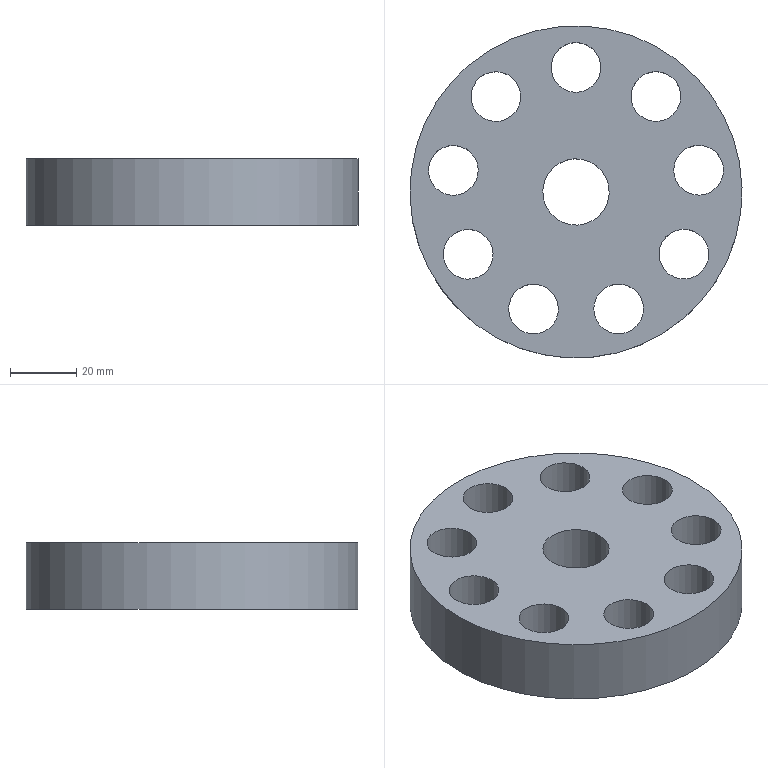Component | NX | CARK1 | 1 solid | 13 faces | box 100 x 100 x 20 mm | volume 118988 mm3 | cylinder 11 | plane 2 | commonest cylinder face diameters 15 x9 20 x1 100 x1
STEP:
#1=CARTESIAN_POINT('',(0.,0.,0.));
#2=DIRECTION('',(0.,0.,1.));
#3=DIRECTION('',(1.,0.,0.));
#4=AXIS2_PLACEMENT_3D('',#1,#2,#3);
#5=CARTESIAN_POINT('',(-1129.876,961.837,201.928));
#6=VERTEX_POINT('',#5);
#7=CARTESIAN_POINT('',(-1123.378,958.091,201.928));
#8=DIRECTION('',(0.,0.,-1.));
#9=DIRECTION('',(-0.8663,0.4995,0.));
#10=AXIS2_PLACEMENT_3D('',#7,#8,#9);
#11=CIRCLE('',#10,7.5);
#12=CARTESIAN_POINT('',(-1123.378,958.091,201.928));
#13=DIRECTION('',(0.,0.,1.));
#14=DIRECTION('',(-0.1743,0.9847,0.));
#15=AXIS2_PLACEMENT_3D('',#12,#13,#14);
#16=CYLINDRICAL_SURFACE('',#15,7.5);
#17=CARTESIAN_POINT('',(7.156,0.));
#18=DIRECTION('',(-1.,0.));
#19=VECTOR('',#18,1.);
#20=LINE('',#17,#19);
#21=(GEOMETRIC_REPRESENTATION_CONTEXT(2)PARAMETRIC_REPRESENTATION_CONTEXT()REPRESENTATION_CONTEXT('',''));
#22=DEFINITIONAL_REPRESENTATION('',(#20),#21);
#23=PCURVE('',#16,#22);
#24=CARTESIAN_POINT('',(-1174.333,980.065,201.928));
#25=DIRECTION('',(0.,0.,-1.));
#26=DIRECTION('',(0.1743,-0.9847,0.));
#27=AXIS2_PLACEMENT_3D('',#24,#25,#26);
#28=PLANE('',#27);
#29=CARTESIAN_POINT('',(30.517,-46.346));
#30=DIRECTION('',(-0.6428,0.766));
#31=AXIS2_PLACEMENT_2D('',#29,#30);
#32=CIRCLE('',#31,7.5);
#33=(GEOMETRIC_REPRESENTATION_CONTEXT(2)PARAMETRIC_REPRESENTATION_CONTEXT()REPRESENTATION_CONTEXT('',''));
#34=DEFINITIONAL_REPRESENTATION('',(#32),#33);
#35=PCURVE('',#28,#34);
#36=SURFACE_CURVE('',#11,(#23,#35),.PCURVE_S1.);
#37=EDGE_CURVE('',#6,#6,#36,.T.);
#38=ORIENTED_EDGE('',*,*,#37,.F.);
#39=CARTESIAN_POINT('',(-1129.876,961.837,221.928));
#40=VERTEX_POINT('',#39);
#41=CARTESIAN_POINT('',(-1129.876,961.837,201.928));
#42=CARTESIAN_POINT('',(-1129.876,961.837,221.928));
#43=B_SPLINE_CURVE_WITH_KNOTS('',1,(#41,#42),.UNSPECIFIED.,.F.,.F.,(2,2),(0.,20.),.PIECEWISE_BEZIER_KNOTS.);
#44=CARTESIAN_POINT('',(7.156,0.));
#45=DIRECTION('',(0.,1.));
#46=VECTOR('',#45,1.);
#47=LINE('',#44,#46);
#48=(GEOMETRIC_REPRESENTATION_CONTEXT(2)PARAMETRIC_REPRESENTATION_CONTEXT()REPRESENTATION_CONTEXT('',''));
#49=DEFINITIONAL_REPRESENTATION('',(#47),#48);
#50=PCURVE('',#16,#49);
#51=CARTESIAN_POINT('',(0.8727,0.));
#52=DIRECTION('',(0.,1.));
#53=VECTOR('',#52,1.);
#54=LINE('',#51,#53);
#55=(GEOMETRIC_REPRESENTATION_CONTEXT(2)PARAMETRIC_REPRESENTATION_CONTEXT()REPRESENTATION_CONTEXT('',''));
#56=DEFINITIONAL_REPRESENTATION('',(#54),#55);
#57=PCURVE('',#16,#56);
#58=SEAM_CURVE('',#43,(#50,#57),.PCURVE_S1.);
#59=EDGE_CURVE('',#6,#40,#58,.T.);
#60=ORIENTED_EDGE('',*,*,#59,.T.);
#61=CARTESIAN_POINT('',(-1123.378,958.091,221.928));
#62=DIRECTION('',(0.,0.,-1.));
#63=DIRECTION('',(-0.8663,0.4995,0.));
#64=AXIS2_PLACEMENT_3D('',#61,#62,#63);
#65=CIRCLE('',#64,7.5);
#66=CARTESIAN_POINT('',(7.156,20.));
#67=DIRECTION('',(-1.,0.));
#68=VECTOR('',#67,1.);
#69=LINE('',#66,#68);
#70=(GEOMETRIC_REPRESENTATION_CONTEXT(2)PARAMETRIC_REPRESENTATION_CONTEXT()REPRESENTATION_CONTEXT('',''));
#71=DEFINITIONAL_REPRESENTATION('',(#69),#70);
#72=PCURVE('',#16,#71);
#73=CARTESIAN_POINT('',(-1174.333,980.065,221.928));
#74=DIRECTION('',(0.,0.,-1.));
#75=DIRECTION('',(0.1743,-0.9847,0.));
#76=AXIS2_PLACEMENT_3D('',#73,#74,#75);
#77=PLANE('',#76);
#78=CARTESIAN_POINT('',(30.517,-46.346));
#79=DIRECTION('',(-0.6428,0.766));
#80=AXIS2_PLACEMENT_2D('',#78,#79);
#81=CIRCLE('',#80,7.5);
#82=(GEOMETRIC_REPRESENTATION_CONTEXT(2)PARAMETRIC_REPRESENTATION_CONTEXT()REPRESENTATION_CONTEXT('',''));
#83=DEFINITIONAL_REPRESENTATION('',(#81),#82);
#84=PCURVE('',#77,#83);
#85=SURFACE_CURVE('',#65,(#72,#84),.PCURVE_S1.);
#86=EDGE_CURVE('',#40,#40,#85,.T.);
#87=ORIENTED_EDGE('',*,*,#86,.T.);
#88=ORIENTED_EDGE('',*,*,#59,.F.);
#89=EDGE_LOOP('',(#38,#60,#87,#88));
#90=FACE_BOUND('',#89,.F.);
#91=ADVANCED_FACE('',(#90),#16,.F.);
#92=CARTESIAN_POINT('',(-1136.597,999.814,201.928));
#93=VERTEX_POINT('',#92);
#94=CARTESIAN_POINT('',(-1131.78,1005.562,201.928));
#95=DIRECTION('',(0.,0.,-1.));
#96=DIRECTION('',(-0.6423,-0.7665,0.));
#97=AXIS2_PLACEMENT_3D('',#94,#95,#96);
#98=CIRCLE('',#97,7.5);
#99=CARTESIAN_POINT('',(-1131.78,1005.562,201.928));
#100=DIRECTION('',(0.,0.,1.));
#101=DIRECTION('',(-0.1743,0.9847,0.));
#102=AXIS2_PLACEMENT_3D('',#99,#100,#101);
#103=CYLINDRICAL_SURFACE('',#102,7.5);
#104=CARTESIAN_POINT('',(8.552,0.));
#105=DIRECTION('',(-1.,0.));
#106=VECTOR('',#105,1.);
#107=LINE('',#104,#106);
#108=(GEOMETRIC_REPRESENTATION_CONTEXT(2)PARAMETRIC_REPRESENTATION_CONTEXT()REPRESENTATION_CONTEXT('',''));
#109=DEFINITIONAL_REPRESENTATION('',(#107),#108);
#110=PCURVE('',#103,#109);
#111=CARTESIAN_POINT('',(-17.692,-46.346));
#112=DIRECTION('',(0.6428,0.766));
#113=AXIS2_PLACEMENT_2D('',#111,#112);
#114=CIRCLE('',#113,7.5);
#115=(GEOMETRIC_REPRESENTATION_CONTEXT(2)PARAMETRIC_REPRESENTATION_CONTEXT()REPRESENTATION_CONTEXT('',''));
#116=DEFINITIONAL_REPRESENTATION('',(#114),#115);
#117=PCURVE('',#28,#116);
#118=SURFACE_CURVE('',#98,(#110,#117),.PCURVE_S1.);
#119=EDGE_CURVE('',#93,#93,#118,.T.);
#120=ORIENTED_EDGE('',*,*,#119,.F.);
#121=CARTESIAN_POINT('',(-1136.597,999.814,221.928));
#122=VERTEX_POINT('',#121);
#123=CARTESIAN_POINT('',(-1136.597,999.814,201.928));
#124=CARTESIAN_POINT('',(-1136.597,999.814,221.928));
#125=B_SPLINE_CURVE_WITH_KNOTS('',1,(#123,#124),.UNSPECIFIED.,.F.,.F.,(2,2),(0.,20.),.PIECEWISE_BEZIER_KNOTS.);
#126=CARTESIAN_POINT('',(8.552,0.));
#127=DIRECTION('',(0.,1.));
#128=VECTOR('',#127,1.);
#129=LINE('',#126,#128);
#130=(GEOMETRIC_REPRESENTATION_CONTEXT(2)PARAMETRIC_REPRESENTATION_CONTEXT()REPRESENTATION_CONTEXT('',''));
#131=DEFINITIONAL_REPRESENTATION('',(#129),#130);
#132=PCURVE('',#103,#131);
#133=CARTESIAN_POINT('',(2.269,0.));
#134=DIRECTION('',(0.,1.));
#135=VECTOR('',#134,1.);
#136=LINE('',#133,#135);
#137=(GEOMETRIC_REPRESENTATION_CONTEXT(2)PARAMETRIC_REPRESENTATION_CONTEXT()REPRESENTATION_CONTEXT('',''));
#138=DEFINITIONAL_REPRESENTATION('',(#136),#137);
#139=PCURVE('',#103,#138);
#140=SEAM_CURVE('',#125,(#132,#139),.PCURVE_S1.);
#141=EDGE_CURVE('',#93,#122,#140,.T.);
#142=ORIENTED_EDGE('',*,*,#141,.T.);
#143=CARTESIAN_POINT('',(-1131.78,1005.562,221.928));
#144=DIRECTION('',(0.,0.,-1.));
#145=DIRECTION('',(-0.6423,-0.7665,0.));
#146=AXIS2_PLACEMENT_3D('',#143,#144,#145);
#147=CIRCLE('',#146,7.5);
#148=CARTESIAN_POINT('',(8.552,20.));
#149=DIRECTION('',(-1.,0.));
#150=VECTOR('',#149,1.);
#151=LINE('',#148,#150);
#152=(GEOMETRIC_REPRESENTATION_CONTEXT(2)PARAMETRIC_REPRESENTATION_CONTEXT()REPRESENTATION_CONTEXT('',''));
#153=DEFINITIONAL_REPRESENTATION('',(#151),#152);
#154=PCURVE('',#103,#153);
#155=CARTESIAN_POINT('',(-17.692,-46.346));
#156=DIRECTION('',(0.6428,0.766));
#157=AXIS2_PLACEMENT_2D('',#155,#156);
#158=CIRCLE('',#157,7.5);
#159=(GEOMETRIC_REPRESENTATION_CONTEXT(2)PARAMETRIC_REPRESENTATION_CONTEXT()REPRESENTATION_CONTEXT('',''));
#160=DEFINITIONAL_REPRESENTATION('',(#158),#159);
#161=PCURVE('',#77,#160);
#162=SURFACE_CURVE('',#147,(#154,#161),.PCURVE_S1.);
#163=EDGE_CURVE('',#122,#122,#162,.T.);
#164=ORIENTED_EDGE('',*,*,#163,.T.);
#165=ORIENTED_EDGE('',*,*,#141,.F.);
#166=EDGE_LOOP('',(#120,#142,#164,#165));
#167=FACE_BOUND('',#166,.F.);
#168=ADVANCED_FACE('',(#167),#103,.F.);
#169=CARTESIAN_POINT('',(-1145.588,948.636,201.928));
#170=VERTEX_POINT('',#169);
#171=CARTESIAN_POINT('',(-1143.018,941.59,201.928));
#172=DIRECTION('',(0.,0.,-1.));
#173=DIRECTION('',(-0.3426,0.9395,0.));
#174=AXIS2_PLACEMENT_3D('',#171,#172,#173);
#175=CIRCLE('',#174,7.5);
#176=CARTESIAN_POINT('',(-1143.018,941.59,201.928));
#177=DIRECTION('',(0.,0.,1.));
#178=DIRECTION('',(-0.1743,0.9847,0.));
#179=AXIS2_PLACEMENT_3D('',#176,#177,#178);
#180=CYLINDRICAL_SURFACE('',#179,7.5);
#181=CARTESIAN_POINT('',(6.458,0.));
#182=DIRECTION('',(-1.,0.));
#183=VECTOR('',#182,1.);
#184=LINE('',#181,#183);
#185=(GEOMETRIC_REPRESENTATION_CONTEXT(2)PARAMETRIC_REPRESENTATION_CONTEXT()REPRESENTATION_CONTEXT('',''));
#186=DEFINITIONAL_REPRESENTATION('',(#184),#185);
#187=PCURVE('',#180,#186);
#188=CARTESIAN_POINT('',(43.343,-24.131));
#189=DIRECTION('',(-0.9848,0.1736));
#190=AXIS2_PLACEMENT_2D('',#188,#189);
#191=CIRCLE('',#190,7.5);
#192=(GEOMETRIC_REPRESENTATION_CONTEXT(2)PARAMETRIC_REPRESENTATION_CONTEXT()REPRESENTATION_CONTEXT('',''));
#193=DEFINITIONAL_REPRESENTATION('',(#191),#192);
#194=PCURVE('',#28,#193);
#195=SURFACE_CURVE('',#175,(#187,#194),.PCURVE_S1.);
#196=EDGE_CURVE('',#170,#170,#195,.T.);
#197=ORIENTED_EDGE('',*,*,#196,.F.);
#198=CARTESIAN_POINT('',(-1145.588,948.636,221.928));
#199=VERTEX_POINT('',#198);
#200=CARTESIAN_POINT('',(-1145.588,948.636,201.928));
#201=CARTESIAN_POINT('',(-1145.588,948.636,221.928));
#202=B_SPLINE_CURVE_WITH_KNOTS('',1,(#200,#201),.UNSPECIFIED.,.F.,.F.,(2,2),(0.,20.),.PIECEWISE_BEZIER_KNOTS.);
#203=CARTESIAN_POINT('',(6.458,0.));
#204=DIRECTION('',(0.,1.));
#205=VECTOR('',#204,1.);
#206=LINE('',#203,#205);
#207=(GEOMETRIC_REPRESENTATION_CONTEXT(2)PARAMETRIC_REPRESENTATION_CONTEXT()REPRESENTATION_CONTEXT('',''));
#208=DEFINITIONAL_REPRESENTATION('',(#206),#207);
#209=PCURVE('',#180,#208);
#210=CARTESIAN_POINT('',(0.1745,0.));
#211=DIRECTION('',(0.,1.));
#212=VECTOR('',#211,1.);
#213=LINE('',#210,#212);
#214=(GEOMETRIC_REPRESENTATION_CONTEXT(2)PARAMETRIC_REPRESENTATION_CONTEXT()REPRESENTATION_CONTEXT('',''));
#215=DEFINITIONAL_REPRESENTATION('',(#213),#214);
#216=PCURVE('',#180,#215);
#217=SEAM_CURVE('',#202,(#209,#216),.PCURVE_S1.);
#218=EDGE_CURVE('',#170,#199,#217,.T.);
#219=ORIENTED_EDGE('',*,*,#218,.T.);
#220=CARTESIAN_POINT('',(-1143.018,941.59,221.928));
#221=DIRECTION('',(0.,0.,-1.));
#222=DIRECTION('',(-0.3426,0.9395,0.));
#223=AXIS2_PLACEMENT_3D('',#220,#221,#222);
#224=CIRCLE('',#223,7.5);
#225=CARTESIAN_POINT('',(6.458,20.));
#226=DIRECTION('',(-1.,0.));
#227=VECTOR('',#226,1.);
#228=LINE('',#225,#227);
#229=(GEOMETRIC_REPRESENTATION_CONTEXT(2)PARAMETRIC_REPRESENTATION_CONTEXT()REPRESENTATION_CONTEXT('',''));
#230=DEFINITIONAL_REPRESENTATION('',(#228),#229);
#231=PCURVE('',#180,#230);
#232=CARTESIAN_POINT('',(43.343,-24.131));
#233=DIRECTION('',(-0.9848,0.1736));
#234=AXIS2_PLACEMENT_2D('',#232,#233);
#235=CIRCLE('',#234,7.5);
#236=(GEOMETRIC_REPRESENTATION_CONTEXT(2)PARAMETRIC_REPRESENTATION_CONTEXT()REPRESENTATION_CONTEXT('',''));
#237=DEFINITIONAL_REPRESENTATION('',(#235),#236);
#238=PCURVE('',#77,#237);
#239=SURFACE_CURVE('',#224,(#231,#238),.PCURVE_S1.);
#240=EDGE_CURVE('',#199,#199,#239,.T.);
#241=ORIENTED_EDGE('',*,*,#240,.T.);
#242=ORIENTED_EDGE('',*,*,#218,.F.);
#243=EDGE_LOOP('',(#197,#219,#241,#242));
#244=FACE_BOUND('',#243,.F.);
#245=ADVANCED_FACE('',(#244),#180,.F.);
#246=CARTESIAN_POINT('',(-1155.885,1006.821,201.928));
#247=VERTEX_POINT('',#246);
#248=CARTESIAN_POINT('',(-1155.89,1014.321,201.928));
#249=DIRECTION('',(0.,0.,-1.));
#250=DIRECTION('',(0.0006313,-1.,0.));
#251=AXIS2_PLACEMENT_3D('',#248,#249,#250);
#252=CIRCLE('',#251,7.5);
#253=CARTESIAN_POINT('',(-1155.89,1014.321,201.928));
#254=DIRECTION('',(0.,0.,1.));
#255=DIRECTION('',(-0.1743,0.9847,0.));
#256=AXIS2_PLACEMENT_3D('',#253,#254,#255);
#257=CYLINDRICAL_SURFACE('',#256,7.5);
#258=CARTESIAN_POINT('',(9.25,0.));
#259=DIRECTION('',(-1.,0.));
#260=VECTOR('',#259,1.);
#261=LINE('',#258,#260);
#262=(GEOMETRIC_REPRESENTATION_CONTEXT(2)PARAMETRIC_REPRESENTATION_CONTEXT()REPRESENTATION_CONTEXT('',''));
#263=DEFINITIONAL_REPRESENTATION('',(#261),#262);
#264=PCURVE('',#257,#263);
#265=CARTESIAN_POINT('',(-30.517,-24.131));
#266=DIRECTION('',(0.9848,0.1736));
#267=AXIS2_PLACEMENT_2D('',#265,#266);
#268=CIRCLE('',#267,7.5);
#269=(GEOMETRIC_REPRESENTATION_CONTEXT(2)PARAMETRIC_REPRESENTATION_CONTEXT()REPRESENTATION_CONTEXT('',''));
#270=DEFINITIONAL_REPRESENTATION('',(#268),#269);
#271=PCURVE('',#28,#270);
#272=SURFACE_CURVE('',#252,(#264,#271),.PCURVE_S1.);
#273=EDGE_CURVE('',#247,#247,#272,.T.);
#274=ORIENTED_EDGE('',*,*,#273,.F.);
#275=CARTESIAN_POINT('',(-1155.885,1006.821,221.928));
#276=VERTEX_POINT('',#275);
#277=CARTESIAN_POINT('',(-1155.885,1006.821,201.928));
#278=CARTESIAN_POINT('',(-1155.885,1006.821,221.928));
#279=B_SPLINE_CURVE_WITH_KNOTS('',1,(#277,#278),.UNSPECIFIED.,.F.,.F.,(2,2),(0.,20.),.PIECEWISE_BEZIER_KNOTS.);
#280=CARTESIAN_POINT('',(9.25,0.));
#281=DIRECTION('',(0.,1.));
#282=VECTOR('',#281,1.);
#283=LINE('',#280,#282);
#284=(GEOMETRIC_REPRESENTATION_CONTEXT(2)PARAMETRIC_REPRESENTATION_CONTEXT()REPRESENTATION_CONTEXT('',''));
#285=DEFINITIONAL_REPRESENTATION('',(#283),#284);
#286=PCURVE('',#257,#285);
#287=CARTESIAN_POINT('',(2.967,0.));
#288=DIRECTION('',(0.,1.));
#289=VECTOR('',#288,1.);
#290=LINE('',#287,#289);
#291=(GEOMETRIC_REPRESENTATION_CONTEXT(2)PARAMETRIC_REPRESENTATION_CONTEXT()REPRESENTATION_CONTEXT('',''));
#292=DEFINITIONAL_REPRESENTATION('',(#290),#291);
#293=PCURVE('',#257,#292);
#294=SEAM_CURVE('',#279,(#286,#293),.PCURVE_S1.);
#295=EDGE_CURVE('',#247,#276,#294,.T.);
#296=ORIENTED_EDGE('',*,*,#295,.T.);
#297=CARTESIAN_POINT('',(-1155.89,1014.321,221.928));
#298=DIRECTION('',(0.,0.,-1.));
#299=DIRECTION('',(0.0006313,-1.,0.));
#300=AXIS2_PLACEMENT_3D('',#297,#298,#299);
#301=CIRCLE('',#300,7.5);
#302=CARTESIAN_POINT('',(9.25,20.));
#303=DIRECTION('',(-1.,0.));
#304=VECTOR('',#303,1.);
#305=LINE('',#302,#304);
#306=(GEOMETRIC_REPRESENTATION_CONTEXT(2)PARAMETRIC_REPRESENTATION_CONTEXT()REPRESENTATION_CONTEXT('',''));
#307=DEFINITIONAL_REPRESENTATION('',(#305),#306);
#308=PCURVE('',#257,#307);
#309=CARTESIAN_POINT('',(-30.517,-24.131));
#310=DIRECTION('',(0.9848,0.1736));
#311=AXIS2_PLACEMENT_2D('',#309,#310);
#312=CIRCLE('',#311,7.5);
#313=(GEOMETRIC_REPRESENTATION_CONTEXT(2)PARAMETRIC_REPRESENTATION_CONTEXT()REPRESENTATION_CONTEXT('',''));
#314=DEFINITIONAL_REPRESENTATION('',(#312),#313);
#315=PCURVE('',#77,#314);
#316=SURFACE_CURVE('',#301,(#308,#315),.PCURVE_S1.);
#317=EDGE_CURVE('',#276,#276,#316,.T.);
#318=ORIENTED_EDGE('',*,*,#317,.T.);
#319=ORIENTED_EDGE('',*,*,#295,.F.);
#320=EDGE_LOOP('',(#274,#296,#318,#319));
#321=FACE_BOUND('',#320,.F.);
#322=ADVANCED_FACE('',(#321),#257,.F.);
#323=CARTESIAN_POINT('',(-1165.713,975.078,201.928));
#324=VERTEX_POINT('',#323);
#325=CARTESIAN_POINT('',(-1155.866,976.821,201.928));
#326=DIRECTION('',(0.,0.,-1.));
#327=DIRECTION('',(-0.9847,-0.1743,0.));
#328=AXIS2_PLACEMENT_3D('',#325,#326,#327);
#329=CIRCLE('',#328,10.);
#330=CARTESIAN_POINT('',(-1155.866,976.821,201.928));
#331=DIRECTION('',(0.,0.,1.));
#332=DIRECTION('',(-0.1743,0.9847,0.));
#333=AXIS2_PLACEMENT_3D('',#330,#331,#332);
#334=CYLINDRICAL_SURFACE('',#333,10.);
#335=CARTESIAN_POINT('',(7.854,0.));
#336=DIRECTION('',(-1.,0.));
#337=VECTOR('',#336,1.);
#338=LINE('',#335,#337);
#339=(GEOMETRIC_REPRESENTATION_CONTEXT(2)PARAMETRIC_REPRESENTATION_CONTEXT()REPRESENTATION_CONTEXT('',''));
#340=DEFINITIONAL_REPRESENTATION('',(#338),#339);
#341=PCURVE('',#334,#340);
#342=CARTESIAN_POINT('',(6.413,-17.619));
#343=DIRECTION('',(0.,1.));
#344=AXIS2_PLACEMENT_2D('',#342,#343);
#345=CIRCLE('',#344,10.);
#346=(GEOMETRIC_REPRESENTATION_CONTEXT(2)PARAMETRIC_REPRESENTATION_CONTEXT()REPRESENTATION_CONTEXT('',''));
#347=DEFINITIONAL_REPRESENTATION('',(#345),#346);
#348=PCURVE('',#28,#347);
#349=SURFACE_CURVE('',#329,(#341,#348),.PCURVE_S1.);
#350=EDGE_CURVE('',#324,#324,#349,.T.);
#351=ORIENTED_EDGE('',*,*,#350,.F.);
#352=CARTESIAN_POINT('',(-1165.713,975.078,221.928));
#353=VERTEX_POINT('',#352);
#354=CARTESIAN_POINT('',(-1165.713,975.078,201.928));
#355=CARTESIAN_POINT('',(-1165.713,975.078,221.928));
#356=B_SPLINE_CURVE_WITH_KNOTS('',1,(#354,#355),.UNSPECIFIED.,.F.,.F.,(2,2),(0.,20.),.PIECEWISE_BEZIER_KNOTS.);
#357=CARTESIAN_POINT('',(7.854,0.));
#358=DIRECTION('',(0.,1.));
#359=VECTOR('',#358,1.);
#360=LINE('',#357,#359);
#361=(GEOMETRIC_REPRESENTATION_CONTEXT(2)PARAMETRIC_REPRESENTATION_CONTEXT()REPRESENTATION_CONTEXT('',''));
#362=DEFINITIONAL_REPRESENTATION('',(#360),#361);
#363=PCURVE('',#334,#362);
#364=CARTESIAN_POINT('',(1.571,0.));
#365=DIRECTION('',(0.,1.));
#366=VECTOR('',#365,1.);
#367=LINE('',#364,#366);
#368=(GEOMETRIC_REPRESENTATION_CONTEXT(2)PARAMETRIC_REPRESENTATION_CONTEXT()REPRESENTATION_CONTEXT('',''));
#369=DEFINITIONAL_REPRESENTATION('',(#367),#368);
#370=PCURVE('',#334,#369);
#371=SEAM_CURVE('',#356,(#363,#370),.PCURVE_S1.);
#372=EDGE_CURVE('',#324,#353,#371,.T.);
#373=ORIENTED_EDGE('',*,*,#372,.T.);
#374=CARTESIAN_POINT('',(-1155.866,976.821,221.928));
#375=DIRECTION('',(0.,0.,-1.));
#376=DIRECTION('',(-0.9847,-0.1743,0.));
#377=AXIS2_PLACEMENT_3D('',#374,#375,#376);
#378=CIRCLE('',#377,10.);
#379=CARTESIAN_POINT('',(7.854,20.));
#380=DIRECTION('',(-1.,0.));
#381=VECTOR('',#380,1.);
#382=LINE('',#379,#381);
#383=(GEOMETRIC_REPRESENTATION_CONTEXT(2)PARAMETRIC_REPRESENTATION_CONTEXT()REPRESENTATION_CONTEXT('',''));
#384=DEFINITIONAL_REPRESENTATION('',(#382),#383);
#385=PCURVE('',#334,#384);
#386=CARTESIAN_POINT('',(6.413,-17.619));
#387=DIRECTION('',(0.,1.));
#388=AXIS2_PLACEMENT_2D('',#386,#387);
#389=CIRCLE('',#388,10.);
#390=(GEOMETRIC_REPRESENTATION_CONTEXT(2)PARAMETRIC_REPRESENTATION_CONTEXT()REPRESENTATION_CONTEXT('',''));
#391=DEFINITIONAL_REPRESENTATION('',(#389),#390);
#392=PCURVE('',#77,#391);
#393=SURFACE_CURVE('',#378,(#385,#392),.PCURVE_S1.);
#394=EDGE_CURVE('',#353,#353,#393,.T.);
#395=ORIENTED_EDGE('',*,*,#394,.T.);
#396=ORIENTED_EDGE('',*,*,#372,.F.);
#397=EDGE_LOOP('',(#351,#373,#395,#396));
#398=FACE_BOUND('',#397,.F.);
#399=ADVANCED_FACE('',(#398),#334,.F.);
#400=CARTESIAN_POINT('',(-1166.109,948.623,201.928));
#401=VERTEX_POINT('',#400);
#402=CARTESIAN_POINT('',(-1168.67,941.574,201.928));
#403=DIRECTION('',(0.,0.,-1.));
#404=DIRECTION('',(0.3414,0.9399,0.));
#405=AXIS2_PLACEMENT_3D('',#402,#403,#404);
#406=CIRCLE('',#405,7.5);
#407=CARTESIAN_POINT('',(-1168.67,941.574,201.928));
#408=DIRECTION('',(0.,0.,1.));
#409=DIRECTION('',(-0.1743,0.9847,0.));
#410=AXIS2_PLACEMENT_3D('',#407,#408,#409);
#411=CYLINDRICAL_SURFACE('',#410,7.5);
#412=CARTESIAN_POINT('',(12.043,0.));
#413=DIRECTION('',(-1.,0.));
#414=VECTOR('',#413,1.);
#415=LINE('',#412,#414);
#416=(GEOMETRIC_REPRESENTATION_CONTEXT(2)PARAMETRIC_REPRESENTATION_CONTEXT()REPRESENTATION_CONTEXT('',''));
#417=DEFINITIONAL_REPRESENTATION('',(#415),#416);
#418=PCURVE('',#411,#417);
#419=CARTESIAN_POINT('',(38.889,1.131));
#420=DIRECTION('',(-0.866,-0.5));
#421=AXIS2_PLACEMENT_2D('',#419,#420);
#422=CIRCLE('',#421,7.5);
#423=(GEOMETRIC_REPRESENTATION_CONTEXT(2)PARAMETRIC_REPRESENTATION_CONTEXT()REPRESENTATION_CONTEXT('',''));
#424=DEFINITIONAL_REPRESENTATION('',(#422),#423);
#425=PCURVE('',#28,#424);
#426=SURFACE_CURVE('',#406,(#418,#425),.PCURVE_S1.);
#427=EDGE_CURVE('',#401,#401,#426,.T.);
#428=ORIENTED_EDGE('',*,*,#427,.F.);
#429=CARTESIAN_POINT('',(-1166.109,948.623,221.928));
#430=VERTEX_POINT('',#429);
#431=CARTESIAN_POINT('',(-1166.109,948.623,201.928));
#432=CARTESIAN_POINT('',(-1166.109,948.623,221.928));
#433=B_SPLINE_CURVE_WITH_KNOTS('',1,(#431,#432),.UNSPECIFIED.,.F.,.F.,(2,2),(0.,20.),.PIECEWISE_BEZIER_KNOTS.);
#434=CARTESIAN_POINT('',(12.043,0.));
#435=DIRECTION('',(0.,1.));
#436=VECTOR('',#435,1.);
#437=LINE('',#434,#436);
#438=(GEOMETRIC_REPRESENTATION_CONTEXT(2)PARAMETRIC_REPRESENTATION_CONTEXT()REPRESENTATION_CONTEXT('',''));
#439=DEFINITIONAL_REPRESENTATION('',(#437),#438);
#440=PCURVE('',#411,#439);
#441=CARTESIAN_POINT('',(5.76,0.));
#442=DIRECTION('',(0.,1.));
#443=VECTOR('',#442,1.);
#444=LINE('',#441,#443);
#445=(GEOMETRIC_REPRESENTATION_CONTEXT(2)PARAMETRIC_REPRESENTATION_CONTEXT()REPRESENTATION_CONTEXT('',''));
#446=DEFINITIONAL_REPRESENTATION('',(#444),#445);
#447=PCURVE('',#411,#446);
#448=SEAM_CURVE('',#433,(#440,#447),.PCURVE_S1.);
#449=EDGE_CURVE('',#401,#430,#448,.T.);
#450=ORIENTED_EDGE('',*,*,#449,.T.);
#451=CARTESIAN_POINT('',(-1168.67,941.574,221.928));
#452=DIRECTION('',(0.,0.,-1.));
#453=DIRECTION('',(0.3414,0.9399,0.));
#454=AXIS2_PLACEMENT_3D('',#451,#452,#453);
#455=CIRCLE('',#454,7.5);
#456=CARTESIAN_POINT('',(12.043,20.));
#457=DIRECTION('',(-1.,0.));
#458=VECTOR('',#457,1.);
#459=LINE('',#456,#458);
#460=(GEOMETRIC_REPRESENTATION_CONTEXT(2)PARAMETRIC_REPRESENTATION_CONTEXT()REPRESENTATION_CONTEXT('',''));
#461=DEFINITIONAL_REPRESENTATION('',(#459),#460);
#462=PCURVE('',#411,#461);
#463=CARTESIAN_POINT('',(38.889,1.131));
#464=DIRECTION('',(-0.866,-0.5));
#465=AXIS2_PLACEMENT_2D('',#463,#464);
#466=CIRCLE('',#465,7.5);
#467=(GEOMETRIC_REPRESENTATION_CONTEXT(2)PARAMETRIC_REPRESENTATION_CONTEXT()REPRESENTATION_CONTEXT('',''));
#468=DEFINITIONAL_REPRESENTATION('',(#466),#467);
#469=PCURVE('',#77,#468);
#470=SURFACE_CURVE('',#455,(#462,#469),.PCURVE_S1.);
#471=EDGE_CURVE('',#430,#430,#470,.T.);
#472=ORIENTED_EDGE('',*,*,#471,.T.);
#473=ORIENTED_EDGE('',*,*,#449,.F.);
#474=EDGE_LOOP('',(#428,#450,#472,#473));
#475=FACE_BOUND('',#474,.F.);
#476=ADVANCED_FACE('',(#475),#411,.F.);
#477=CARTESIAN_POINT('',(-1175.164,999.79,201.928));
#478=VERTEX_POINT('',#477);
#479=CARTESIAN_POINT('',(-1179.989,1005.532,201.928));
#480=DIRECTION('',(0.,0.,-1.));
#481=DIRECTION('',(0.6433,-0.7656,0.));
#482=AXIS2_PLACEMENT_3D('',#479,#480,#481);
#483=CIRCLE('',#482,7.5);
#484=CARTESIAN_POINT('',(-1179.989,1005.532,201.928));
#485=DIRECTION('',(0.,0.,1.));
#486=DIRECTION('',(-0.1743,0.9847,0.));
#487=AXIS2_PLACEMENT_3D('',#484,#485,#486);
#488=CYLINDRICAL_SURFACE('',#487,7.5);
#489=CARTESIAN_POINT('',(9.948,0.));
#490=DIRECTION('',(-1.,0.));
#491=VECTOR('',#490,1.);
#492=LINE('',#489,#491);
#493=(GEOMETRIC_REPRESENTATION_CONTEXT(2)PARAMETRIC_REPRESENTATION_CONTEXT()REPRESENTATION_CONTEXT('',''));
#494=DEFINITIONAL_REPRESENTATION('',(#492),#493);
#495=PCURVE('',#488,#494);
#496=CARTESIAN_POINT('',(-26.063,1.131));
#497=DIRECTION('',(0.866,-0.5));
#498=AXIS2_PLACEMENT_2D('',#496,#497);
#499=CIRCLE('',#498,7.5);
#500=(GEOMETRIC_REPRESENTATION_CONTEXT(2)PARAMETRIC_REPRESENTATION_CONTEXT()REPRESENTATION_CONTEXT('',''));
#501=DEFINITIONAL_REPRESENTATION('',(#499),#500);
#502=PCURVE('',#28,#501);
#503=SURFACE_CURVE('',#483,(#495,#502),.PCURVE_S1.);
#504=EDGE_CURVE('',#478,#478,#503,.T.);
#505=ORIENTED_EDGE('',*,*,#504,.F.);
#506=CARTESIAN_POINT('',(-1175.164,999.79,221.928));
#507=VERTEX_POINT('',#506);
#508=CARTESIAN_POINT('',(-1175.164,999.79,201.928));
#509=CARTESIAN_POINT('',(-1175.164,999.79,221.928));
#510=B_SPLINE_CURVE_WITH_KNOTS('',1,(#508,#509),.UNSPECIFIED.,.F.,.F.,(2,2),(0.,20.),.PIECEWISE_BEZIER_KNOTS.);
#511=CARTESIAN_POINT('',(9.948,0.));
#512=DIRECTION('',(0.,1.));
#513=VECTOR('',#512,1.);
#514=LINE('',#511,#513);
#515=(GEOMETRIC_REPRESENTATION_CONTEXT(2)PARAMETRIC_REPRESENTATION_CONTEXT()REPRESENTATION_CONTEXT('',''));
#516=DEFINITIONAL_REPRESENTATION('',(#514),#515);
#517=PCURVE('',#488,#516);
#518=CARTESIAN_POINT('',(3.665,0.));
#519=DIRECTION('',(0.,1.));
#520=VECTOR('',#519,1.);
#521=LINE('',#518,#520);
#522=(GEOMETRIC_REPRESENTATION_CONTEXT(2)PARAMETRIC_REPRESENTATION_CONTEXT()REPRESENTATION_CONTEXT('',''));
#523=DEFINITIONAL_REPRESENTATION('',(#521),#522);
#524=PCURVE('',#488,#523);
#525=SEAM_CURVE('',#510,(#517,#524),.PCURVE_S1.);
#526=EDGE_CURVE('',#478,#507,#525,.T.);
#527=ORIENTED_EDGE('',*,*,#526,.T.);
#528=CARTESIAN_POINT('',(-1179.989,1005.532,221.928));
#529=DIRECTION('',(0.,0.,-1.));
#530=DIRECTION('',(0.6433,-0.7656,0.));
#531=AXIS2_PLACEMENT_3D('',#528,#529,#530);
#532=CIRCLE('',#531,7.5);
#533=CARTESIAN_POINT('',(9.948,20.));
#534=DIRECTION('',(-1.,0.));
#535=VECTOR('',#534,1.);
#536=LINE('',#533,#535);
#537=(GEOMETRIC_REPRESENTATION_CONTEXT(2)PARAMETRIC_REPRESENTATION_CONTEXT()REPRESENTATION_CONTEXT('',''));
#538=DEFINITIONAL_REPRESENTATION('',(#536),#537);
#539=PCURVE('',#488,#538);
#540=CARTESIAN_POINT('',(-26.063,1.131));
#541=DIRECTION('',(0.866,-0.5));
#542=AXIS2_PLACEMENT_2D('',#540,#541);
#543=CIRCLE('',#542,7.5);
#544=(GEOMETRIC_REPRESENTATION_CONTEXT(2)PARAMETRIC_REPRESENTATION_CONTEXT()REPRESENTATION_CONTEXT('',''));
#545=DEFINITIONAL_REPRESENTATION('',(#543),#544);
#546=PCURVE('',#77,#545);
#547=SURFACE_CURVE('',#532,(#539,#546),.PCURVE_S1.);
#548=EDGE_CURVE('',#507,#507,#547,.T.);
#549=ORIENTED_EDGE('',*,*,#548,.T.);
#550=ORIENTED_EDGE('',*,*,#526,.F.);
#551=EDGE_LOOP('',(#505,#527,#549,#550));
#552=FACE_BOUND('',#551,.F.);
#553=ADVANCED_FACE('',(#552),#488,.F.);
#554=CARTESIAN_POINT('',(-1181.837,961.804,201.928));
#555=VERTEX_POINT('',#554);
#556=CARTESIAN_POINT('',(-1188.33,958.05,201.928));
#557=DIRECTION('',(0.,0.,-1.));
#558=DIRECTION('',(0.8657,0.5005,0.));
#559=AXIS2_PLACEMENT_3D('',#556,#557,#558);
#560=CIRCLE('',#559,7.5);
#561=CARTESIAN_POINT('',(-1188.33,958.05,201.928));
#562=DIRECTION('',(0.,0.,1.));
#563=DIRECTION('',(-0.1743,0.9847,0.));
#564=AXIS2_PLACEMENT_3D('',#561,#562,#563);
#565=CYLINDRICAL_SURFACE('',#564,7.5);
#566=CARTESIAN_POINT('',(11.345,0.));
#567=DIRECTION('',(-1.,0.));
#568=VECTOR('',#567,1.);
#569=LINE('',#566,#568);
#570=(GEOMETRIC_REPRESENTATION_CONTEXT(2)PARAMETRIC_REPRESENTATION_CONTEXT()REPRESENTATION_CONTEXT('',''));
#571=DEFINITIONAL_REPRESENTATION('',(#569),#570);
#572=PCURVE('',#565,#571);
#573=CARTESIAN_POINT('',(19.239,17.619));
#574=DIRECTION('',(-0.342,-0.9397));
#575=AXIS2_PLACEMENT_2D('',#573,#574);
#576=CIRCLE('',#575,7.5);
#577=(GEOMETRIC_REPRESENTATION_CONTEXT(2)PARAMETRIC_REPRESENTATION_CONTEXT()REPRESENTATION_CONTEXT('',''));
#578=DEFINITIONAL_REPRESENTATION('',(#576),#577);
#579=PCURVE('',#28,#578);
#580=SURFACE_CURVE('',#560,(#572,#579),.PCURVE_S1.);
#581=EDGE_CURVE('',#555,#555,#580,.T.);
#582=ORIENTED_EDGE('',*,*,#581,.F.);
#583=CARTESIAN_POINT('',(-1181.837,961.804,221.928));
#584=VERTEX_POINT('',#583);
#585=CARTESIAN_POINT('',(-1181.837,961.804,201.928));
#586=CARTESIAN_POINT('',(-1181.837,961.804,221.928));
#587=B_SPLINE_CURVE_WITH_KNOTS('',1,(#585,#586),.UNSPECIFIED.,.F.,.F.,(2,2),(0.,20.),.PIECEWISE_BEZIER_KNOTS.);
#588=CARTESIAN_POINT('',(11.345,0.));
#589=DIRECTION('',(0.,1.));
#590=VECTOR('',#589,1.);
#591=LINE('',#588,#590);
#592=(GEOMETRIC_REPRESENTATION_CONTEXT(2)PARAMETRIC_REPRESENTATION_CONTEXT()REPRESENTATION_CONTEXT('',''));
#593=DEFINITIONAL_REPRESENTATION('',(#591),#592);
#594=PCURVE('',#565,#593);
#595=CARTESIAN_POINT('',(5.061,0.));
#596=DIRECTION('',(0.,1.));
#597=VECTOR('',#596,1.);
#598=LINE('',#595,#597);
#599=(GEOMETRIC_REPRESENTATION_CONTEXT(2)PARAMETRIC_REPRESENTATION_CONTEXT()REPRESENTATION_CONTEXT('',''));
#600=DEFINITIONAL_REPRESENTATION('',(#598),#599);
#601=PCURVE('',#565,#600);
#602=SEAM_CURVE('',#587,(#594,#601),.PCURVE_S1.);
#603=EDGE_CURVE('',#555,#584,#602,.T.);
#604=ORIENTED_EDGE('',*,*,#603,.T.);
#605=CARTESIAN_POINT('',(-1188.33,958.05,221.928));
#606=DIRECTION('',(0.,0.,-1.));
#607=DIRECTION('',(0.8657,0.5005,0.));
#608=AXIS2_PLACEMENT_3D('',#605,#606,#607);
#609=CIRCLE('',#608,7.5);
#610=CARTESIAN_POINT('',(11.345,20.));
#611=DIRECTION('',(-1.,0.));
#612=VECTOR('',#611,1.);
#613=LINE('',#610,#612);
#614=(GEOMETRIC_REPRESENTATION_CONTEXT(2)PARAMETRIC_REPRESENTATION_CONTEXT()REPRESENTATION_CONTEXT('',''));
#615=DEFINITIONAL_REPRESENTATION('',(#613),#614);
#616=PCURVE('',#565,#615);
#617=CARTESIAN_POINT('',(19.239,17.619));
#618=DIRECTION('',(-0.342,-0.9397));
#619=AXIS2_PLACEMENT_2D('',#617,#618);
#620=CIRCLE('',#619,7.5);
#621=(GEOMETRIC_REPRESENTATION_CONTEXT(2)PARAMETRIC_REPRESENTATION_CONTEXT()REPRESENTATION_CONTEXT('',''));
#622=DEFINITIONAL_REPRESENTATION('',(#620),#621);
#623=PCURVE('',#77,#622);
#624=SURFACE_CURVE('',#609,(#616,#623),.PCURVE_S1.);
#625=EDGE_CURVE('',#584,#584,#624,.T.);
#626=ORIENTED_EDGE('',*,*,#625,.T.);
#627=ORIENTED_EDGE('',*,*,#603,.F.);
#628=EDGE_LOOP('',(#582,#604,#626,#627));
#629=FACE_BOUND('',#628,.F.);
#630=ADVANCED_FACE('',(#629),#565,.F.);
#631=CARTESIAN_POINT('',(-1185.414,982.011,201.928));
#632=VERTEX_POINT('',#631);
#633=CARTESIAN_POINT('',(-1192.8,983.309,201.928));
#634=DIRECTION('',(0.,0.,-1.));
#635=DIRECTION('',(0.9849,-0.173,0.));
#636=AXIS2_PLACEMENT_3D('',#633,#634,#635);
#637=CIRCLE('',#636,7.5);
#638=CARTESIAN_POINT('',(-1192.8,983.309,201.928));
#639=DIRECTION('',(0.,0.,1.));
#640=DIRECTION('',(-0.1743,0.9847,0.));
#641=AXIS2_PLACEMENT_3D('',#638,#639,#640);
#642=CYLINDRICAL_SURFACE('',#641,7.5);
#643=CARTESIAN_POINT('',(10.647,0.));
#644=DIRECTION('',(-1.,0.));
#645=VECTOR('',#644,1.);
#646=LINE('',#643,#645);
#647=(GEOMETRIC_REPRESENTATION_CONTEXT(2)PARAMETRIC_REPRESENTATION_CONTEXT()REPRESENTATION_CONTEXT('',''));
#648=DEFINITIONAL_REPRESENTATION('',(#646),#647);
#649=PCURVE('',#642,#648);
#650=CARTESIAN_POINT('',(-6.413,17.619));
#651=DIRECTION('',(0.342,-0.9397));
#652=AXIS2_PLACEMENT_2D('',#650,#651);
#653=CIRCLE('',#652,7.5);
#654=(GEOMETRIC_REPRESENTATION_CONTEXT(2)PARAMETRIC_REPRESENTATION_CONTEXT()REPRESENTATION_CONTEXT('',''));
#655=DEFINITIONAL_REPRESENTATION('',(#653),#654);
#656=PCURVE('',#28,#655);
#657=SURFACE_CURVE('',#637,(#649,#656),.PCURVE_S1.);
#658=EDGE_CURVE('',#632,#632,#657,.T.);
#659=ORIENTED_EDGE('',*,*,#658,.F.);
#660=CARTESIAN_POINT('',(-1185.414,982.011,221.928));
#661=VERTEX_POINT('',#660);
#662=CARTESIAN_POINT('',(-1185.414,982.011,201.928));
#663=CARTESIAN_POINT('',(-1185.414,982.011,221.928));
#664=B_SPLINE_CURVE_WITH_KNOTS('',1,(#662,#663),.UNSPECIFIED.,.F.,.F.,(2,2),(0.,20.),.PIECEWISE_BEZIER_KNOTS.);
#665=CARTESIAN_POINT('',(10.647,0.));
#666=DIRECTION('',(0.,1.));
#667=VECTOR('',#666,1.);
#668=LINE('',#665,#667);
#669=(GEOMETRIC_REPRESENTATION_CONTEXT(2)PARAMETRIC_REPRESENTATION_CONTEXT()REPRESENTATION_CONTEXT('',''));
#670=DEFINITIONAL_REPRESENTATION('',(#668),#669);
#671=PCURVE('',#642,#670);
#672=CARTESIAN_POINT('',(4.363,0.));
#673=DIRECTION('',(0.,1.));
#674=VECTOR('',#673,1.);
#675=LINE('',#672,#674);
#676=(GEOMETRIC_REPRESENTATION_CONTEXT(2)PARAMETRIC_REPRESENTATION_CONTEXT()REPRESENTATION_CONTEXT('',''));
#677=DEFINITIONAL_REPRESENTATION('',(#675),#676);
#678=PCURVE('',#642,#677);
#679=SEAM_CURVE('',#664,(#671,#678),.PCURVE_S1.);
#680=EDGE_CURVE('',#632,#661,#679,.T.);
#681=ORIENTED_EDGE('',*,*,#680,.T.);
#682=CARTESIAN_POINT('',(-1192.8,983.309,221.928));
#683=DIRECTION('',(0.,0.,-1.));
#684=DIRECTION('',(0.9849,-0.173,0.));
#685=AXIS2_PLACEMENT_3D('',#682,#683,#684);
#686=CIRCLE('',#685,7.5);
#687=CARTESIAN_POINT('',(10.647,20.));
#688=DIRECTION('',(-1.,0.));
#689=VECTOR('',#688,1.);
#690=LINE('',#687,#689);
#691=(GEOMETRIC_REPRESENTATION_CONTEXT(2)PARAMETRIC_REPRESENTATION_CONTEXT()REPRESENTATION_CONTEXT('',''));
#692=DEFINITIONAL_REPRESENTATION('',(#690),#691);
#693=PCURVE('',#642,#692);
#694=CARTESIAN_POINT('',(-6.413,17.619));
#695=DIRECTION('',(0.342,-0.9397));
#696=AXIS2_PLACEMENT_2D('',#694,#695);
#697=CIRCLE('',#696,7.5);
#698=(GEOMETRIC_REPRESENTATION_CONTEXT(2)PARAMETRIC_REPRESENTATION_CONTEXT()REPRESENTATION_CONTEXT('',''));
#699=DEFINITIONAL_REPRESENTATION('',(#697),#698);
#700=PCURVE('',#77,#699);
#701=SURFACE_CURVE('',#686,(#693,#700),.PCURVE_S1.);
#702=EDGE_CURVE('',#661,#661,#701,.T.);
#703=ORIENTED_EDGE('',*,*,#702,.T.);
#704=ORIENTED_EDGE('',*,*,#680,.F.);
#705=EDGE_LOOP('',(#659,#681,#703,#704));
#706=FACE_BOUND('',#705,.F.);
#707=ADVANCED_FACE('',(#706),#642,.F.);
#708=CARTESIAN_POINT('',(-1205.101,968.107,201.928));
#709=VERTEX_POINT('',#708);
#710=CARTESIAN_POINT('',(-1155.866,976.821,201.928));
#711=DIRECTION('',(0.,0.,-1.));
#712=DIRECTION('',(-0.9847,-0.1743,0.));
#713=AXIS2_PLACEMENT_3D('',#710,#711,#712);
#714=CIRCLE('',#713,50.);
#715=CARTESIAN_POINT('',(-1155.866,976.821,201.928));
#716=DIRECTION('',(0.,0.,1.));
#717=DIRECTION('',(-0.1743,0.9847,0.));
#718=AXIS2_PLACEMENT_3D('',#715,#716,#717);
#719=CYLINDRICAL_SURFACE('',#718,50.);
#720=CARTESIAN_POINT('',(7.854,0.));
#721=DIRECTION('',(-1.,0.));
#722=VECTOR('',#721,1.);
#723=LINE('',#720,#722);
#724=(GEOMETRIC_REPRESENTATION_CONTEXT(2)PARAMETRIC_REPRESENTATION_CONTEXT()REPRESENTATION_CONTEXT('',''));
#725=DEFINITIONAL_REPRESENTATION('',(#723),#724);
#726=PCURVE('',#719,#725);
#727=CARTESIAN_POINT('',(6.413,-17.619));
#728=DIRECTION('',(-0.,1.));
#729=AXIS2_PLACEMENT_2D('',#727,#728);
#730=CIRCLE('',#729,50.);
#731=(GEOMETRIC_REPRESENTATION_CONTEXT(2)PARAMETRIC_REPRESENTATION_CONTEXT()REPRESENTATION_CONTEXT('',''));
#732=DEFINITIONAL_REPRESENTATION('',(#730),#731);
#733=PCURVE('',#28,#732);
#734=SURFACE_CURVE('',#714,(#726,#733),.PCURVE_S1.);
#735=EDGE_CURVE('',#709,#709,#734,.T.);
#736=ORIENTED_EDGE('',*,*,#735,.F.);
#737=CARTESIAN_POINT('',(-1205.101,968.107,221.928));
#738=VERTEX_POINT('',#737);
#739=CARTESIAN_POINT('',(-1205.101,968.107,201.928));
#740=CARTESIAN_POINT('',(-1205.101,968.107,221.928));
#741=B_SPLINE_CURVE_WITH_KNOTS('',1,(#739,#740),.UNSPECIFIED.,.F.,.F.,(2,2),(0.,20.),.PIECEWISE_BEZIER_KNOTS.);
#742=CARTESIAN_POINT('',(7.854,0.));
#743=DIRECTION('',(0.,1.));
#744=VECTOR('',#743,1.);
#745=LINE('',#742,#744);
#746=(GEOMETRIC_REPRESENTATION_CONTEXT(2)PARAMETRIC_REPRESENTATION_CONTEXT()REPRESENTATION_CONTEXT('',''));
#747=DEFINITIONAL_REPRESENTATION('',(#745),#746);
#748=PCURVE('',#719,#747);
#749=CARTESIAN_POINT('',(1.571,0.));
#750=DIRECTION('',(0.,1.));
#751=VECTOR('',#750,1.);
#752=LINE('',#749,#751);
#753=(GEOMETRIC_REPRESENTATION_CONTEXT(2)PARAMETRIC_REPRESENTATION_CONTEXT()REPRESENTATION_CONTEXT('',''));
#754=DEFINITIONAL_REPRESENTATION('',(#752),#753);
#755=PCURVE('',#719,#754);
#756=SEAM_CURVE('',#741,(#748,#755),.PCURVE_S1.);
#757=EDGE_CURVE('',#709,#738,#756,.T.);
#758=ORIENTED_EDGE('',*,*,#757,.T.);
#759=CARTESIAN_POINT('',(-1155.866,976.821,221.928));
#760=DIRECTION('',(0.,0.,-1.));
#761=DIRECTION('',(-0.9847,-0.1743,0.));
#762=AXIS2_PLACEMENT_3D('',#759,#760,#761);
#763=CIRCLE('',#762,50.);
#764=CARTESIAN_POINT('',(7.854,20.));
#765=DIRECTION('',(-1.,0.));
#766=VECTOR('',#765,1.);
#767=LINE('',#764,#766);
#768=(GEOMETRIC_REPRESENTATION_CONTEXT(2)PARAMETRIC_REPRESENTATION_CONTEXT()REPRESENTATION_CONTEXT('',''));
#769=DEFINITIONAL_REPRESENTATION('',(#767),#768);
#770=PCURVE('',#719,#769);
#771=CARTESIAN_POINT('',(6.413,-17.619));
#772=DIRECTION('',(-0.,1.));
#773=AXIS2_PLACEMENT_2D('',#771,#772);
#774=CIRCLE('',#773,50.);
#775=(GEOMETRIC_REPRESENTATION_CONTEXT(2)PARAMETRIC_REPRESENTATION_CONTEXT()REPRESENTATION_CONTEXT('',''));
#776=DEFINITIONAL_REPRESENTATION('',(#774),#775);
#777=PCURVE('',#77,#776);
#778=SURFACE_CURVE('',#763,(#770,#777),.PCURVE_S1.);
#779=EDGE_CURVE('',#738,#738,#778,.T.);
#780=ORIENTED_EDGE('',*,*,#779,.T.);
#781=ORIENTED_EDGE('',*,*,#757,.F.);
#782=EDGE_LOOP('',(#736,#758,#780,#781));
#783=FACE_BOUND('',#782,.T.);
#784=ADVANCED_FACE('',(#783),#719,.T.);
#785=CARTESIAN_POINT('',(-1126.325,982.049,201.928));
#786=VERTEX_POINT('',#785);
#787=CARTESIAN_POINT('',(-1118.94,983.356,201.928));
#788=DIRECTION('',(0.,0.,-1.));
#789=DIRECTION('',(-0.9847,-0.1743,0.));
#790=AXIS2_PLACEMENT_3D('',#787,#788,#789);
#791=CIRCLE('',#790,7.5);
#792=CARTESIAN_POINT('',(-1118.94,983.356,201.928));
#793=DIRECTION('',(0.,0.,1.));
#794=DIRECTION('',(-0.1743,0.9847,0.));
#795=AXIS2_PLACEMENT_3D('',#792,#793,#794);
#796=CYLINDRICAL_SURFACE('',#795,7.5);
#797=CARTESIAN_POINT('',(7.854,0.));
#798=DIRECTION('',(-1.,0.));
#799=VECTOR('',#798,1.);
#800=LINE('',#797,#799);
#801=(GEOMETRIC_REPRESENTATION_CONTEXT(2)PARAMETRIC_REPRESENTATION_CONTEXT()REPRESENTATION_CONTEXT('',''));
#802=DEFINITIONAL_REPRESENTATION('',(#800),#801);
#803=PCURVE('',#796,#802);
#804=CARTESIAN_POINT('',(6.413,-55.119));
#805=DIRECTION('',(0.,1.));
#806=AXIS2_PLACEMENT_2D('',#804,#805);
#807=CIRCLE('',#806,7.5);
#808=(GEOMETRIC_REPRESENTATION_CONTEXT(2)PARAMETRIC_REPRESENTATION_CONTEXT()REPRESENTATION_CONTEXT('',''));
#809=DEFINITIONAL_REPRESENTATION('',(#807),#808);
#810=PCURVE('',#28,#809);
#811=SURFACE_CURVE('',#791,(#803,#810),.PCURVE_S1.);
#812=EDGE_CURVE('',#786,#786,#811,.T.);
#813=ORIENTED_EDGE('',*,*,#812,.F.);
#814=CARTESIAN_POINT('',(-1126.325,982.049,221.928));
#815=VERTEX_POINT('',#814);
#816=CARTESIAN_POINT('',(-1126.325,982.049,201.928));
#817=CARTESIAN_POINT('',(-1126.325,982.049,221.928));
#818=B_SPLINE_CURVE_WITH_KNOTS('',1,(#816,#817),.UNSPECIFIED.,.F.,.F.,(2,2),(0.,20.),.PIECEWISE_BEZIER_KNOTS.);
#819=CARTESIAN_POINT('',(7.854,0.));
#820=DIRECTION('',(0.,1.));
#821=VECTOR('',#820,1.);
#822=LINE('',#819,#821);
#823=(GEOMETRIC_REPRESENTATION_CONTEXT(2)PARAMETRIC_REPRESENTATION_CONTEXT()REPRESENTATION_CONTEXT('',''));
#824=DEFINITIONAL_REPRESENTATION('',(#822),#823);
#825=PCURVE('',#796,#824);
#826=CARTESIAN_POINT('',(1.571,0.));
#827=DIRECTION('',(0.,1.));
#828=VECTOR('',#827,1.);
#829=LINE('',#826,#828);
#830=(GEOMETRIC_REPRESENTATION_CONTEXT(2)PARAMETRIC_REPRESENTATION_CONTEXT()REPRESENTATION_CONTEXT('',''));
#831=DEFINITIONAL_REPRESENTATION('',(#829),#830);
#832=PCURVE('',#796,#831);
#833=SEAM_CURVE('',#818,(#825,#832),.PCURVE_S1.);
#834=EDGE_CURVE('',#786,#815,#833,.T.);
#835=ORIENTED_EDGE('',*,*,#834,.T.);
#836=CARTESIAN_POINT('',(-1118.94,983.356,221.928));
#837=DIRECTION('',(0.,0.,-1.));
#838=DIRECTION('',(-0.9847,-0.1743,0.));
#839=AXIS2_PLACEMENT_3D('',#836,#837,#838);
#840=CIRCLE('',#839,7.5);
#841=CARTESIAN_POINT('',(7.854,20.));
#842=DIRECTION('',(-1.,0.));
#843=VECTOR('',#842,1.);
#844=LINE('',#841,#843);
#845=(GEOMETRIC_REPRESENTATION_CONTEXT(2)PARAMETRIC_REPRESENTATION_CONTEXT()REPRESENTATION_CONTEXT('',''));
#846=DEFINITIONAL_REPRESENTATION('',(#844),#845);
#847=PCURVE('',#796,#846);
#848=CARTESIAN_POINT('',(6.413,-55.119));
#849=DIRECTION('',(0.,1.));
#850=AXIS2_PLACEMENT_2D('',#848,#849);
#851=CIRCLE('',#850,7.5);
#852=(GEOMETRIC_REPRESENTATION_CONTEXT(2)PARAMETRIC_REPRESENTATION_CONTEXT()REPRESENTATION_CONTEXT('',''));
#853=DEFINITIONAL_REPRESENTATION('',(#851),#852);
#854=PCURVE('',#77,#853);
#855=SURFACE_CURVE('',#840,(#847,#854),.PCURVE_S1.);
#856=EDGE_CURVE('',#815,#815,#855,.T.);
#857=ORIENTED_EDGE('',*,*,#856,.T.);
#858=ORIENTED_EDGE('',*,*,#834,.F.);
#859=EDGE_LOOP('',(#813,#835,#857,#858));
#860=FACE_BOUND('',#859,.F.);
#861=ADVANCED_FACE('',(#860),#796,.F.);
#862=ORIENTED_EDGE('',*,*,#735,.T.);
#863=EDGE_LOOP('',(#862));
#864=FACE_BOUND('',#863,.T.);
#865=ORIENTED_EDGE('',*,*,#658,.F.);
#866=EDGE_LOOP('',(#865));
#867=FACE_BOUND('',#866,.T.);
#868=ORIENTED_EDGE('',*,*,#581,.F.);
#869=EDGE_LOOP('',(#868));
#870=FACE_BOUND('',#869,.T.);
#871=ORIENTED_EDGE('',*,*,#504,.F.);
#872=EDGE_LOOP('',(#871));
#873=FACE_BOUND('',#872,.T.);
#874=ORIENTED_EDGE('',*,*,#427,.F.);
#875=EDGE_LOOP('',(#874));
#876=FACE_BOUND('',#875,.T.);
#877=ORIENTED_EDGE('',*,*,#350,.F.);
#878=EDGE_LOOP('',(#877));
#879=FACE_BOUND('',#878,.T.);
#880=ORIENTED_EDGE('',*,*,#273,.F.);
#881=EDGE_LOOP('',(#880));
#882=FACE_BOUND('',#881,.T.);
#883=ORIENTED_EDGE('',*,*,#196,.F.);
#884=EDGE_LOOP('',(#883));
#885=FACE_BOUND('',#884,.T.);
#886=ORIENTED_EDGE('',*,*,#119,.F.);
#887=EDGE_LOOP('',(#886));
#888=FACE_BOUND('',#887,.T.);
#889=ORIENTED_EDGE('',*,*,#37,.F.);
#890=EDGE_LOOP('',(#889));
#891=FACE_BOUND('',#890,.T.);
#892=ORIENTED_EDGE('',*,*,#812,.F.);
#893=EDGE_LOOP('',(#892));
#894=FACE_BOUND('',#893,.T.);
#895=ADVANCED_FACE('',(#864,#867,#870,#873,#876,#879,#882,#885,#888,#891,#894),#28,.T.);
#896=ORIENTED_EDGE('',*,*,#779,.F.);
#897=EDGE_LOOP('',(#896));
#898=FACE_BOUND('',#897,.T.);
#899=ORIENTED_EDGE('',*,*,#702,.T.);
#900=EDGE_LOOP('',(#899));
#901=FACE_BOUND('',#900,.T.);
#902=ORIENTED_EDGE('',*,*,#625,.T.);
#903=EDGE_LOOP('',(#902));
#904=FACE_BOUND('',#903,.T.);
#905=ORIENTED_EDGE('',*,*,#548,.T.);
#906=EDGE_LOOP('',(#905));
#907=FACE_BOUND('',#906,.T.);
#908=ORIENTED_EDGE('',*,*,#471,.T.);
#909=EDGE_LOOP('',(#908));
#910=FACE_BOUND('',#909,.T.);
#911=ORIENTED_EDGE('',*,*,#394,.T.);
#912=EDGE_LOOP('',(#911));
#913=FACE_BOUND('',#912,.T.);
#914=ORIENTED_EDGE('',*,*,#317,.T.);
#915=EDGE_LOOP('',(#914));
#916=FACE_BOUND('',#915,.T.);
#917=ORIENTED_EDGE('',*,*,#240,.T.);
#918=EDGE_LOOP('',(#917));
#919=FACE_BOUND('',#918,.T.);
#920=ORIENTED_EDGE('',*,*,#163,.T.);
#921=EDGE_LOOP('',(#920));
#922=FACE_BOUND('',#921,.T.);
#923=ORIENTED_EDGE('',*,*,#86,.T.);
#924=EDGE_LOOP('',(#923));
#925=FACE_BOUND('',#924,.T.);
#926=ORIENTED_EDGE('',*,*,#856,.T.);
#927=EDGE_LOOP('',(#926));
#928=FACE_BOUND('',#927,.T.);
#929=ADVANCED_FACE('',(#898,#901,#904,#907,#910,#913,#916,#919,#922,#925,#928),#77,.F.);
#930=CLOSED_SHELL('',(#91,#168,#245,#322,#399,#476,#553,#630,#707,#784,#861,#895,#929));
#931=MANIFOLD_SOLID_BREP('',#930);
#932=(LENGTH_UNIT()NAMED_UNIT(*)SI_UNIT(.MILLI.,.METRE.));
#933=UNCERTAINTY_MEASURE_WITH_UNIT(LENGTH_MEASURE(0.00001),#932,'','');
#934=(NAMED_UNIT(*)PLANE_ANGLE_UNIT()SI_UNIT($,.RADIAN.));
#935=(NAMED_UNIT(*)SI_UNIT($,.STERADIAN.)SOLID_ANGLE_UNIT());
#936=(GEOMETRIC_REPRESENTATION_CONTEXT(3)GLOBAL_UNCERTAINTY_ASSIGNED_CONTEXT((#933))GLOBAL_UNIT_ASSIGNED_CONTEXT((#932,#934,#935))REPRESENTATION_CONTEXT('',''));
#937=ADVANCED_BREP_SHAPE_REPRESENTATION('',(#4,#931),#936);